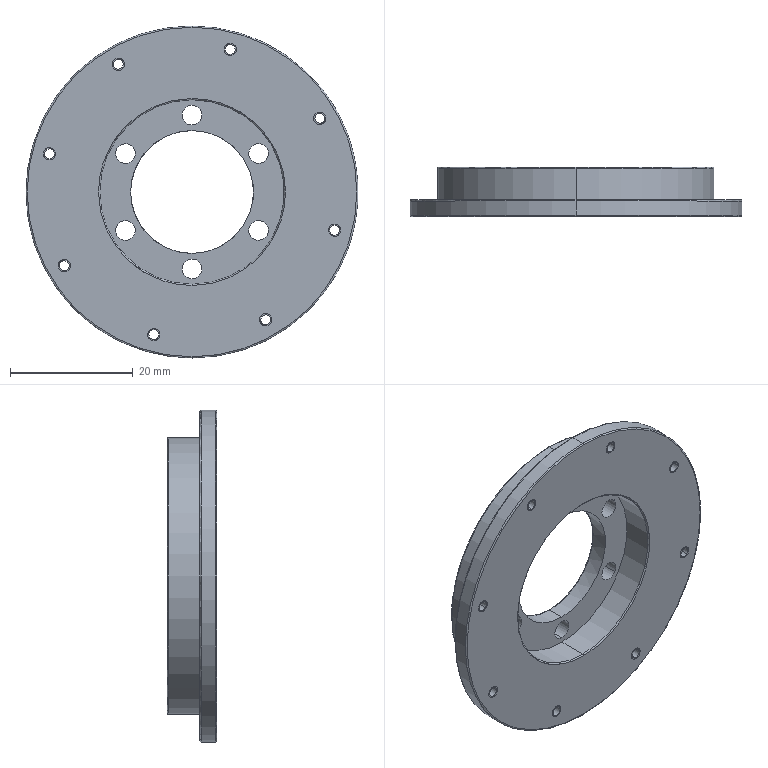CAM job | Mastercam | mm | 1 operations | part box 54 x 8 x 54
1. Drill/Counterbore | 1 - 2 倒角刀